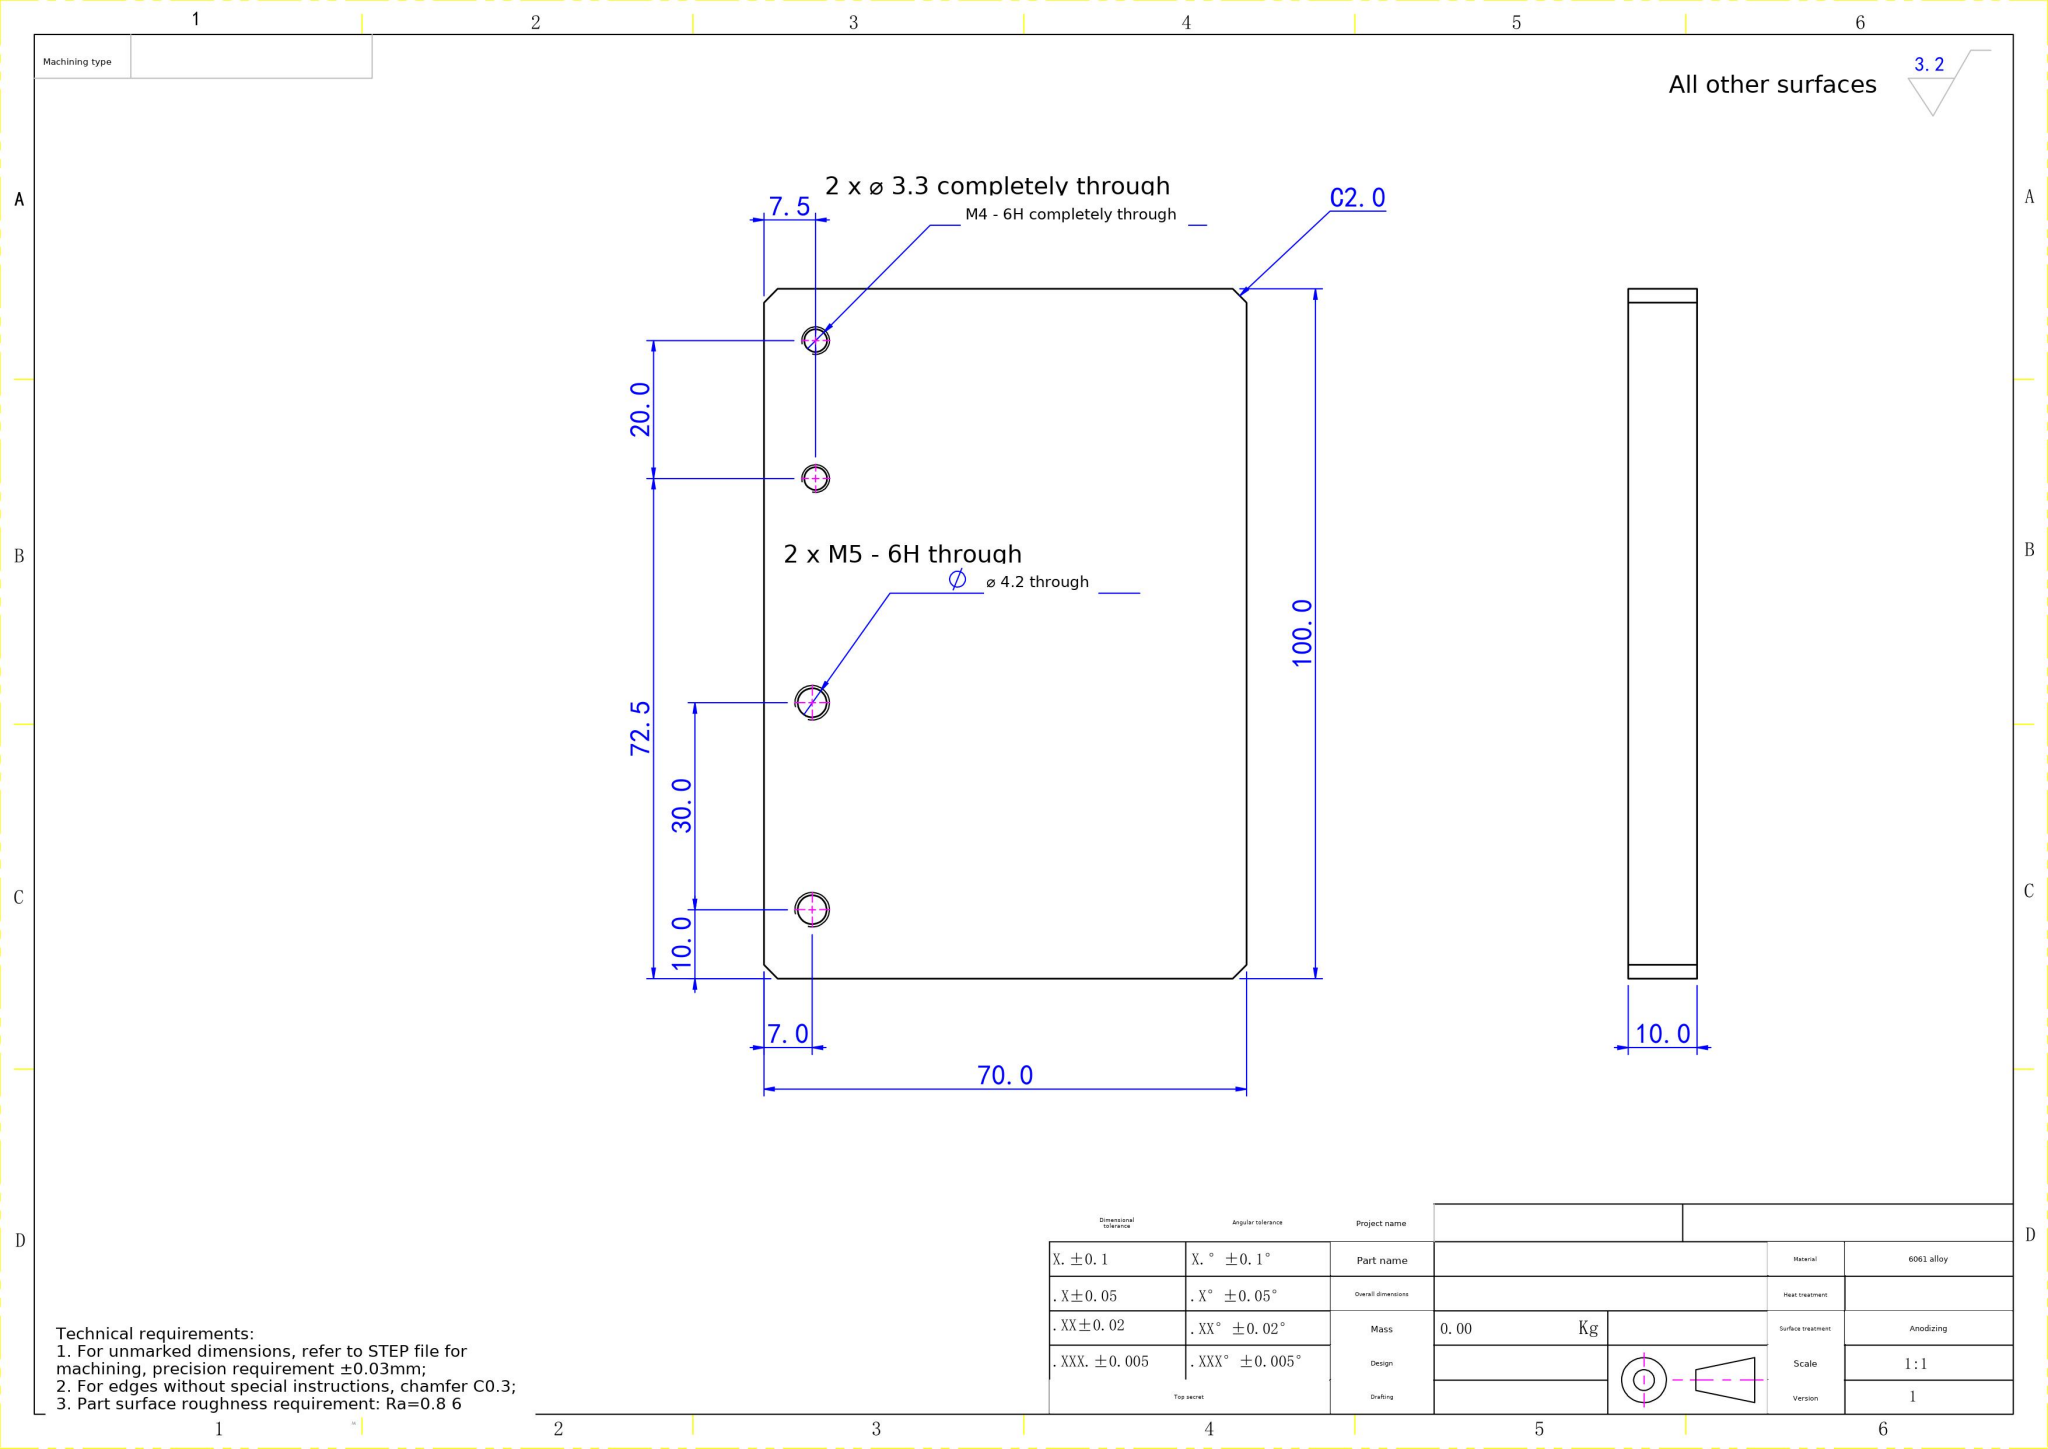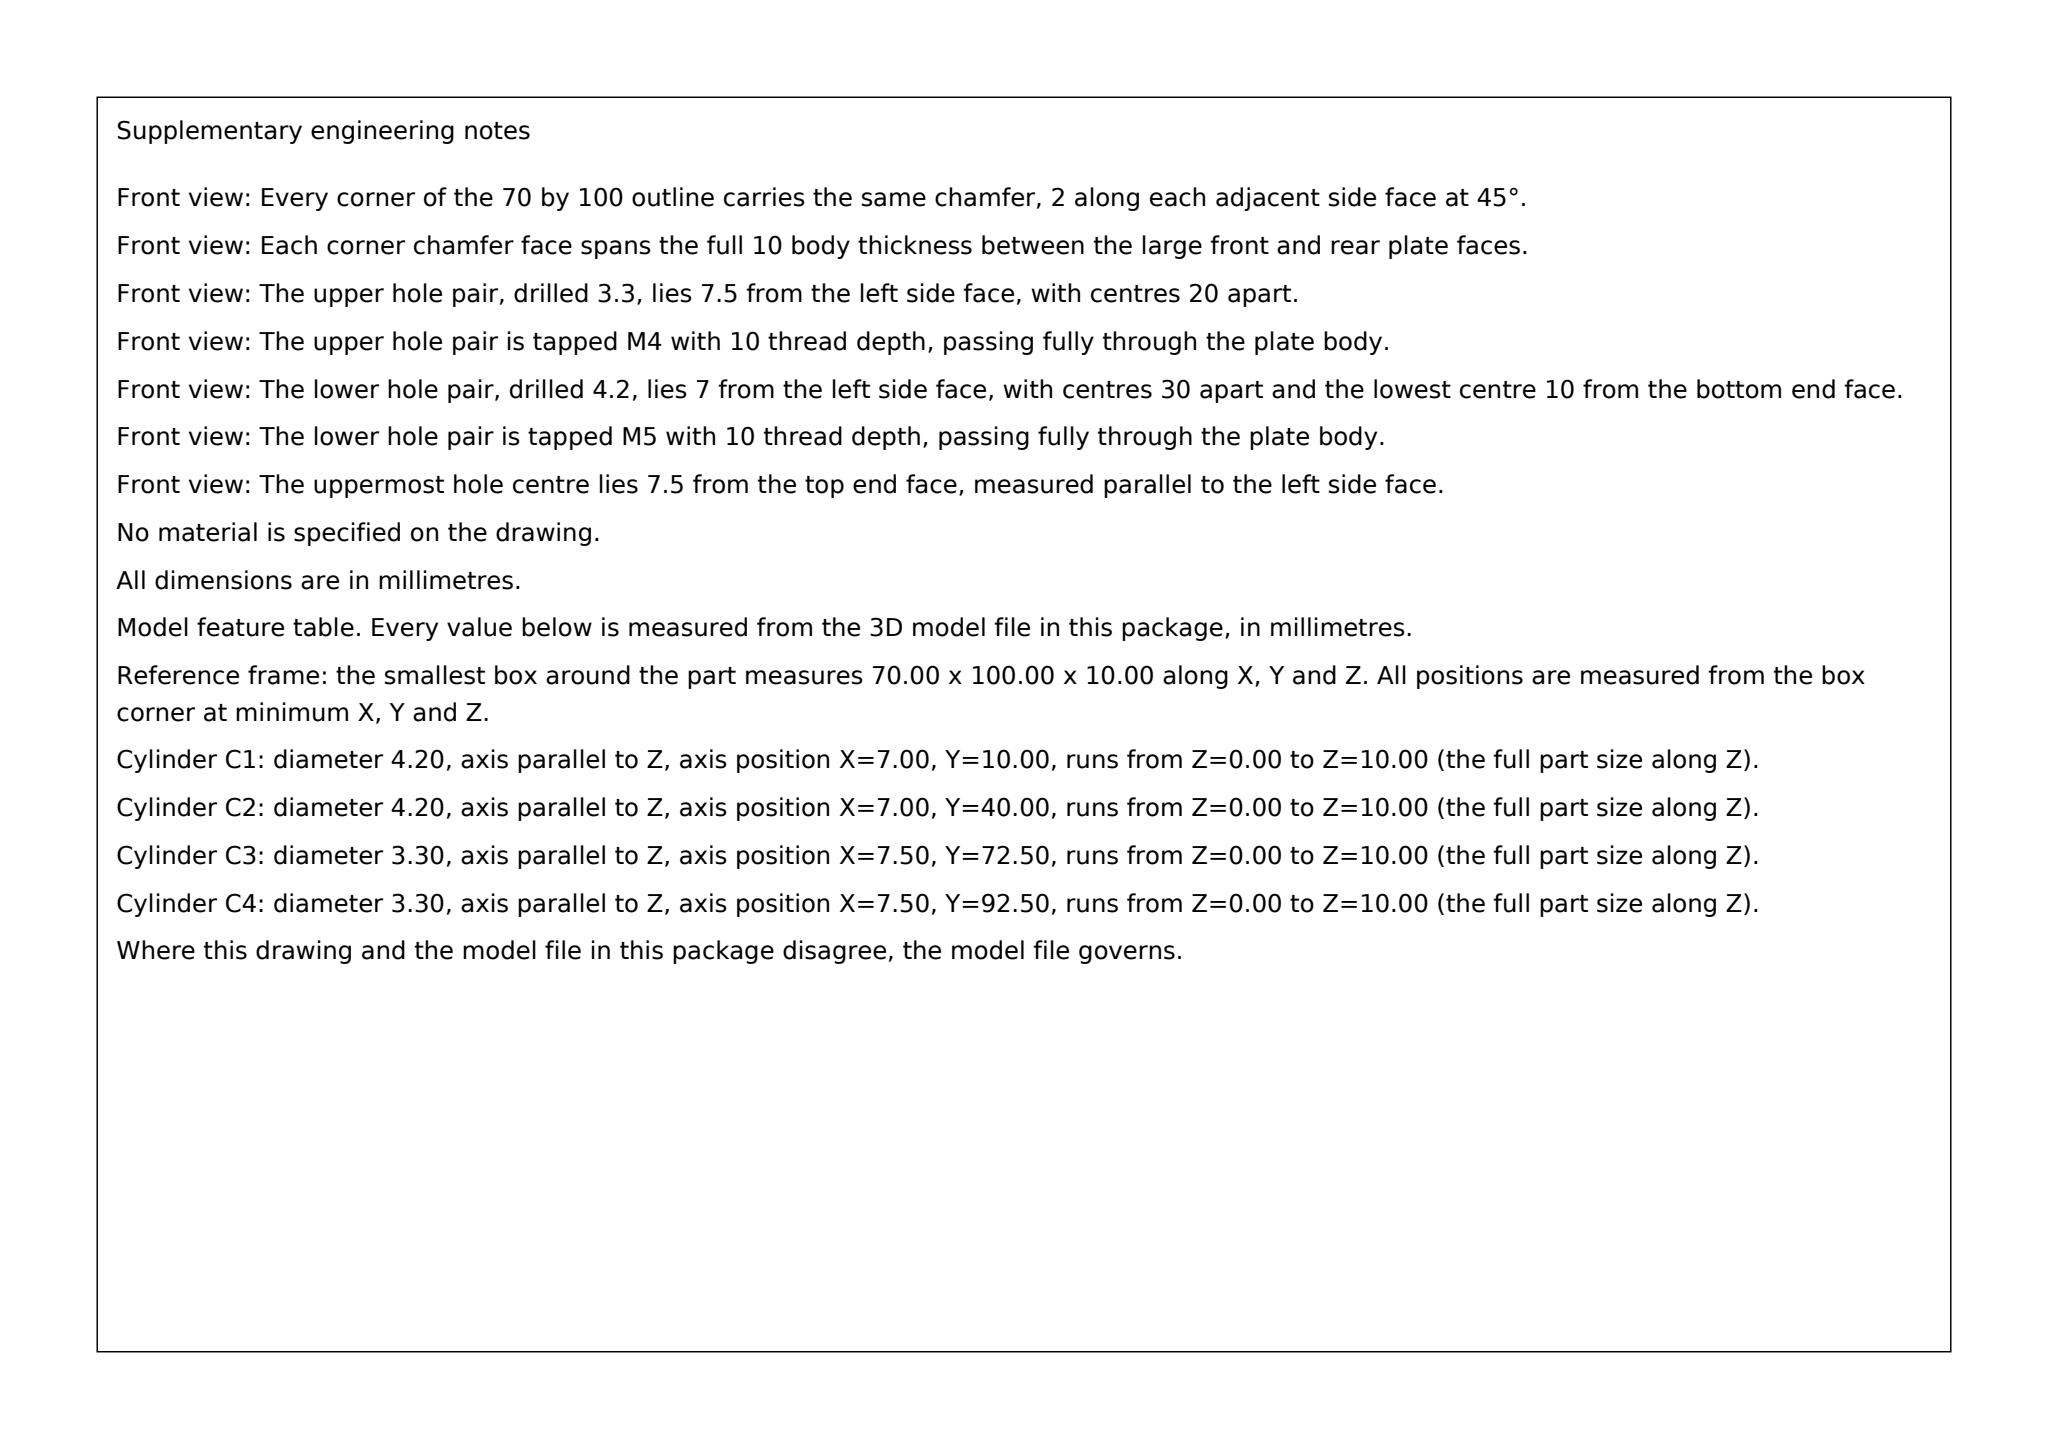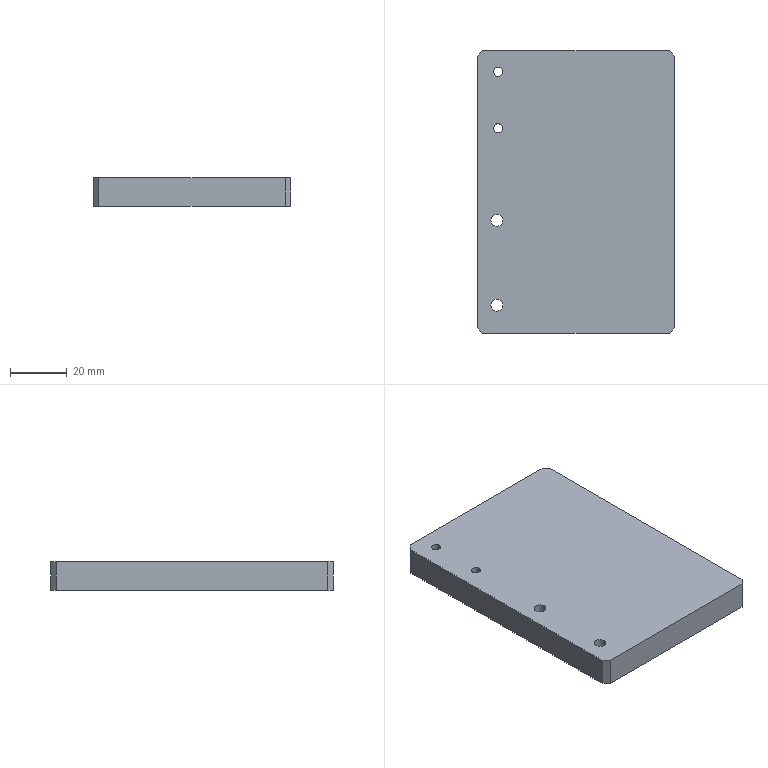Part | SolidWorks | mm | material 6061 alloy | 1 solid | 18 faces | box 70 x 100 x 10 mm | volume 69472 mm3 | plane 10 | cylinder 8 | commonest cylinder face diameters 4.2 x4 3.3 x4
build123d program:
from build123d import *

# Parameters (mm, degrees)
SKETCH1_W           = 70
SKETCH1_H           = 100
BOSS_EXTRUDE1_DEPTH = 10
M4_TAPPED_HOLE1_D   = 3.3
CHAMFER1_SIZE       = 2
M5_TAPPED_HOLE1_D   = 4.2


with BuildPart() as part:
    # Sketch1 → Boss-Extrude1 (new body)
    with BuildSketch(Plane.XY):
        with Locations((35, 50)):
            Rectangle(SKETCH1_W, SKETCH1_H)
    extrude(amount=BOSS_EXTRUDE1_DEPTH)

    # M4 Tapped Hole1 (through all)
    with Locations(Plane.XY.offset(10)):
        with Locations((7.5, 92.5), (7.5, 72.5)):
            Hole(M4_TAPPED_HOLE1_D / 2)

    # Chamfer1
    chamfer1_edges = [part.edges().sort_by_distance(p)[0] for p in [
        (0, 100, 5),
        (70, 100, 5),
        (70, 0, 5),
        (0, 0, 5),
    ]]
    chamfer(chamfer1_edges, length=CHAMFER1_SIZE)

    # M5 Tapped Hole1 (through all)
    with Locations(Plane.XY.offset(10)):
        with Locations((7, 10), (7, 40)):
            Hole(M5_TAPPED_HOLE1_D / 2)


solid = part.part